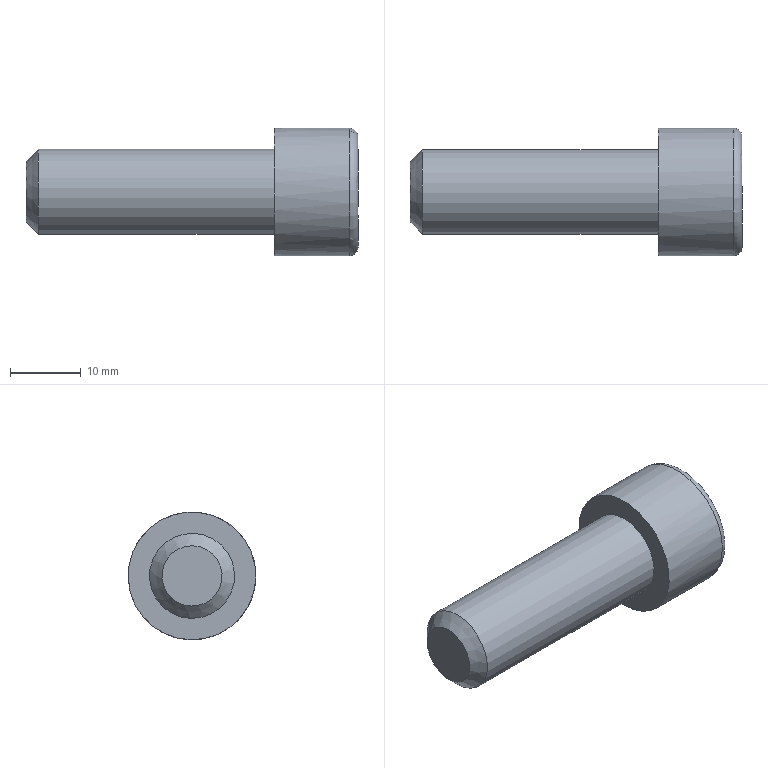Component | NX | 12_03_SCREW_M12X35_DIN912_2 | 1 solid | 14 faces | box 46.8 x 18 x 18 mm | volume 6372 mm3 | plane 10 | cylinder 2 | cone 1 | torus 1 | commonest cylinder face diameters 12 x1 18 x1
STEP:
#1=CARTESIAN_POINT('',(0.,0.,0.));
#2=DIRECTION('',(0.,0.,1.));
#3=DIRECTION('',(1.,0.,0.));
#4=AXIS2_PLACEMENT_3D('',#1,#2,#3);
#5=CARTESIAN_POINT('',(30.8,27.791,32.022));
#6=VERTEX_POINT('',#5);
#7=CARTESIAN_POINT('',(30.8,35.,35.));
#8=DIRECTION('',(1.,0.,0.));
#9=DIRECTION('',(0.,-0.9242,-0.3818));
#10=AXIS2_PLACEMENT_3D('',#7,#8,#9);
#11=CIRCLE('',#10,7.8);
#12=CARTESIAN_POINT('',(30.8,43.318,38.437));
#13=DIRECTION('',(-1.,-0.,-0.));
#14=DIRECTION('',(0.,-0.9242,-0.3818));
#15=AXIS2_PLACEMENT_3D('',#12,#13,#14);
#16=PLANE('',#15);
#17=CARTESIAN_POINT('',(16.8,0.));
#18=CARTESIAN_POINT('',(16.8,-13.51));
#19=CARTESIAN_POINT('',(5.1,-6.755));
#20=CARTESIAN_POINT('',(-6.6,0.));
#21=CARTESIAN_POINT('',(5.1,6.755));
#22=CARTESIAN_POINT('',(16.8,13.51));
#23=CARTESIAN_POINT('',(16.8,0.));
#24=(BOUNDED_CURVE()B_SPLINE_CURVE(2,(#17,#18,#19,#20,#21,#22,#23),.UNSPECIFIED.,.T.,.F.)B_SPLINE_CURVE_WITH_KNOTS((1,2,2,2,2,1),(-2.094,0.,2.094,4.189,6.283,8.378),.UNSPECIFIED.)CURVE()GEOMETRIC_REPRESENTATION_ITEM()RATIONAL_B_SPLINE_CURVE((1.,0.5,1.,0.5,1.,0.5,1.))REPRESENTATION_ITEM(''));
#25=(GEOMETRIC_REPRESENTATION_CONTEXT(2)PARAMETRIC_REPRESENTATION_CONTEXT()REPRESENTATION_CONTEXT('',''));
#26=DEFINITIONAL_REPRESENTATION('',(#24),#25);
#27=PCURVE('',#16,#26);
#28=CARTESIAN_POINT('',(29.6,35.,35.));
#29=DIRECTION('',(-1.,-0.,-0.));
#30=DIRECTION('',(0.,-0.9242,-0.3818));
#31=AXIS2_PLACEMENT_3D('',#28,#29,#30);
#32=TOROIDAL_SURFACE('',#31,7.8,1.2);
#33=CARTESIAN_POINT('',(6.283,4.712));
#34=DIRECTION('',(-1.,0.));
#35=VECTOR('',#34,1.);
#36=LINE('',#33,#35);
#37=(GEOMETRIC_REPRESENTATION_CONTEXT(2)PARAMETRIC_REPRESENTATION_CONTEXT()REPRESENTATION_CONTEXT('',''));
#38=DEFINITIONAL_REPRESENTATION('',(#36),#37);
#39=PCURVE('',#32,#38);
#40=SURFACE_CURVE('',#11,(#27,#39),.PCURVE_S1.);
#41=EDGE_CURVE('',#6,#6,#40,.T.);
#42=ORIENTED_EDGE('',*,*,#41,.T.);
#43=EDGE_LOOP('',(#42));
#44=FACE_BOUND('',#43,.T.);
#45=CARTESIAN_POINT('',(30.8,39.577,31.481));
#46=VERTEX_POINT('',#45);
#47=CARTESIAN_POINT('',(30.8,40.336,37.205));
#48=VERTEX_POINT('',#47);
#49=CARTESIAN_POINT('',(30.8,39.577,31.481));
#50=DIRECTION('',(0.,0.1314,0.9913));
#51=VECTOR('',#50,1.);
#52=LINE('',#49,#51);
#53=CARTESIAN_POINT('',(6.113,-5.));
#54=DIRECTION('',(-0.5,0.866));
#55=VECTOR('',#54,1.);
#56=LINE('',#53,#55);
#57=(GEOMETRIC_REPRESENTATION_CONTEXT(2)PARAMETRIC_REPRESENTATION_CONTEXT()REPRESENTATION_CONTEXT('',''));
#58=DEFINITIONAL_REPRESENTATION('',(#56),#57);
#59=PCURVE('',#16,#58);
#60=CARTESIAN_POINT('',(24.8,39.577,31.481));
#61=DIRECTION('',(0.,0.9913,-0.1314));
#62=DIRECTION('',(0.,-0.1314,-0.9913));
#63=AXIS2_PLACEMENT_3D('',#60,#61,#62);
#64=PLANE('',#63);
#65=CARTESIAN_POINT('',(0.,-6.));
#66=DIRECTION('',(-1.,0.));
#67=VECTOR('',#66,1.);
#68=LINE('',#65,#67);
#69=(GEOMETRIC_REPRESENTATION_CONTEXT(2)PARAMETRIC_REPRESENTATION_CONTEXT()REPRESENTATION_CONTEXT('',''));
#70=DEFINITIONAL_REPRESENTATION('',(#68),#69);
#71=PCURVE('',#64,#70);
#72=SURFACE_CURVE('',#52,(#59,#71),.PCURVE_S1.);
#73=EDGE_CURVE('',#46,#48,#72,.T.);
#74=ORIENTED_EDGE('',*,*,#73,.F.);
#75=CARTESIAN_POINT('',(30.8,34.241,29.277));
#76=VERTEX_POINT('',#75);
#77=CARTESIAN_POINT('',(30.8,34.241,29.277));
#78=DIRECTION('',(0.,0.9242,0.3818));
#79=VECTOR('',#78,1.);
#80=LINE('',#77,#79);
#81=CARTESIAN_POINT('',(11.887,-5.));
#82=DIRECTION('',(-1.,-0.));
#83=VECTOR('',#82,1.);
#84=LINE('',#81,#83);
#85=(GEOMETRIC_REPRESENTATION_CONTEXT(2)PARAMETRIC_REPRESENTATION_CONTEXT()REPRESENTATION_CONTEXT('',''));
#86=DEFINITIONAL_REPRESENTATION('',(#84),#85);
#87=PCURVE('',#16,#86);
#88=CARTESIAN_POINT('',(24.8,34.241,29.277));
#89=DIRECTION('',(0.,0.3818,-0.9242));
#90=DIRECTION('',(0.,-0.9242,-0.3818));
#91=AXIS2_PLACEMENT_3D('',#88,#89,#90);
#92=PLANE('',#91);
#93=CARTESIAN_POINT('',(0.,-6.));
#94=DIRECTION('',(-1.,0.));
#95=VECTOR('',#94,1.);
#96=LINE('',#93,#95);
#97=(GEOMETRIC_REPRESENTATION_CONTEXT(2)PARAMETRIC_REPRESENTATION_CONTEXT()REPRESENTATION_CONTEXT('',''));
#98=DEFINITIONAL_REPRESENTATION('',(#96),#97);
#99=PCURVE('',#92,#98);
#100=SURFACE_CURVE('',#80,(#87,#99),.PCURVE_S1.);
#101=EDGE_CURVE('',#76,#46,#100,.T.);
#102=ORIENTED_EDGE('',*,*,#101,.F.);
#103=CARTESIAN_POINT('',(30.8,29.664,32.795));
#104=VERTEX_POINT('',#103);
#105=CARTESIAN_POINT('',(30.8,29.664,32.795));
#106=DIRECTION('',(0.,0.7928,-0.6095));
#107=VECTOR('',#106,1.);
#108=LINE('',#105,#107);
#109=CARTESIAN_POINT('',(14.774,0.));
#110=DIRECTION('',(-0.5,-0.866));
#111=VECTOR('',#110,1.);
#112=LINE('',#109,#111);
#113=(GEOMETRIC_REPRESENTATION_CONTEXT(2)PARAMETRIC_REPRESENTATION_CONTEXT()REPRESENTATION_CONTEXT('',''));
#114=DEFINITIONAL_REPRESENTATION('',(#112),#113);
#115=PCURVE('',#16,#114);
#116=CARTESIAN_POINT('',(24.8,29.664,32.795));
#117=DIRECTION('',(0.,-0.6095,-0.7928));
#118=DIRECTION('',(0.,-0.7928,0.6095));
#119=AXIS2_PLACEMENT_3D('',#116,#117,#118);
#120=PLANE('',#119);
#121=CARTESIAN_POINT('',(0.,-6.));
#122=DIRECTION('',(-1.,0.));
#123=VECTOR('',#122,1.);
#124=LINE('',#121,#123);
#125=(GEOMETRIC_REPRESENTATION_CONTEXT(2)PARAMETRIC_REPRESENTATION_CONTEXT()REPRESENTATION_CONTEXT('',''));
#126=DEFINITIONAL_REPRESENTATION('',(#124),#125);
#127=PCURVE('',#120,#126);
#128=SURFACE_CURVE('',#108,(#115,#127),.PCURVE_S1.);
#129=EDGE_CURVE('',#104,#76,#128,.T.);
#130=ORIENTED_EDGE('',*,*,#129,.F.);
#131=CARTESIAN_POINT('',(30.8,30.423,38.519));
#132=VERTEX_POINT('',#131);
#133=CARTESIAN_POINT('',(30.8,30.423,38.519));
#134=DIRECTION('',(0.,-0.1314,-0.9913));
#135=VECTOR('',#134,1.);
#136=LINE('',#133,#135);
#137=CARTESIAN_POINT('',(11.887,5.));
#138=DIRECTION('',(0.5,-0.866));
#139=VECTOR('',#138,1.);
#140=LINE('',#137,#139);
#141=(GEOMETRIC_REPRESENTATION_CONTEXT(2)PARAMETRIC_REPRESENTATION_CONTEXT()REPRESENTATION_CONTEXT('',''));
#142=DEFINITIONAL_REPRESENTATION('',(#140),#141);
#143=PCURVE('',#16,#142);
#144=CARTESIAN_POINT('',(24.8,30.423,38.519));
#145=DIRECTION('',(0.,-0.9913,0.1314));
#146=DIRECTION('',(0.,0.1314,0.9913));
#147=AXIS2_PLACEMENT_3D('',#144,#145,#146);
#148=PLANE('',#147);
#149=CARTESIAN_POINT('',(0.,-6.));
#150=DIRECTION('',(-1.,0.));
#151=VECTOR('',#150,1.);
#152=LINE('',#149,#151);
#153=(GEOMETRIC_REPRESENTATION_CONTEXT(2)PARAMETRIC_REPRESENTATION_CONTEXT()REPRESENTATION_CONTEXT('',''));
#154=DEFINITIONAL_REPRESENTATION('',(#152),#153);
#155=PCURVE('',#148,#154);
#156=SURFACE_CURVE('',#136,(#143,#155),.PCURVE_S1.);
#157=EDGE_CURVE('',#132,#104,#156,.T.);
#158=ORIENTED_EDGE('',*,*,#157,.F.);
#159=CARTESIAN_POINT('',(30.8,35.759,40.723));
#160=VERTEX_POINT('',#159);
#161=CARTESIAN_POINT('',(30.8,35.759,40.723));
#162=DIRECTION('',(0.,-0.9242,-0.3818));
#163=VECTOR('',#162,1.);
#164=LINE('',#161,#163);
#165=CARTESIAN_POINT('',(6.113,5.));
#166=DIRECTION('',(1.,0.));
#167=VECTOR('',#166,1.);
#168=LINE('',#165,#167);
#169=(GEOMETRIC_REPRESENTATION_CONTEXT(2)PARAMETRIC_REPRESENTATION_CONTEXT()REPRESENTATION_CONTEXT('',''));
#170=DEFINITIONAL_REPRESENTATION('',(#168),#169);
#171=PCURVE('',#16,#170);
#172=CARTESIAN_POINT('',(24.8,35.759,40.723));
#173=DIRECTION('',(0.,-0.3818,0.9242));
#174=DIRECTION('',(0.,0.9242,0.3818));
#175=AXIS2_PLACEMENT_3D('',#172,#173,#174);
#176=PLANE('',#175);
#177=CARTESIAN_POINT('',(0.,-6.));
#178=DIRECTION('',(-1.,0.));
#179=VECTOR('',#178,1.);
#180=LINE('',#177,#179);
#181=(GEOMETRIC_REPRESENTATION_CONTEXT(2)PARAMETRIC_REPRESENTATION_CONTEXT()REPRESENTATION_CONTEXT('',''));
#182=DEFINITIONAL_REPRESENTATION('',(#180),#181);
#183=PCURVE('',#176,#182);
#184=SURFACE_CURVE('',#164,(#171,#183),.PCURVE_S1.);
#185=EDGE_CURVE('',#160,#132,#184,.T.);
#186=ORIENTED_EDGE('',*,*,#185,.F.);
#187=CARTESIAN_POINT('',(30.8,40.336,37.205));
#188=DIRECTION('',(0.,-0.7928,0.6095));
#189=VECTOR('',#188,1.);
#190=LINE('',#187,#189);
#191=CARTESIAN_POINT('',(3.226,0.));
#192=DIRECTION('',(0.5,0.866));
#193=VECTOR('',#192,1.);
#194=LINE('',#191,#193);
#195=(GEOMETRIC_REPRESENTATION_CONTEXT(2)PARAMETRIC_REPRESENTATION_CONTEXT()REPRESENTATION_CONTEXT('',''));
#196=DEFINITIONAL_REPRESENTATION('',(#194),#195);
#197=PCURVE('',#16,#196);
#198=CARTESIAN_POINT('',(24.8,40.336,37.205));
#199=DIRECTION('',(0.,0.6095,0.7928));
#200=DIRECTION('',(0.,0.7928,-0.6095));
#201=AXIS2_PLACEMENT_3D('',#198,#199,#200);
#202=PLANE('',#201);
#203=CARTESIAN_POINT('',(0.,-6.));
#204=DIRECTION('',(-1.,0.));
#205=VECTOR('',#204,1.);
#206=LINE('',#203,#205);
#207=(GEOMETRIC_REPRESENTATION_CONTEXT(2)PARAMETRIC_REPRESENTATION_CONTEXT()REPRESENTATION_CONTEXT('',''));
#208=DEFINITIONAL_REPRESENTATION('',(#206),#207);
#209=PCURVE('',#202,#208);
#210=SURFACE_CURVE('',#190,(#197,#209),.PCURVE_S1.);
#211=EDGE_CURVE('',#48,#160,#210,.T.);
#212=ORIENTED_EDGE('',*,*,#211,.F.);
#213=EDGE_LOOP('',(#74,#102,#130,#158,#186,#212));
#214=FACE_BOUND('',#213,.T.);
#215=ADVANCED_FACE('',(#44,#214),#16,.F.);
#216=CARTESIAN_POINT('',(-16.,38.928,36.623));
#217=VERTEX_POINT('',#216);
#218=CARTESIAN_POINT('',(-16.,35.,35.));
#219=DIRECTION('',(-1.,-0.,-0.));
#220=DIRECTION('',(-0.,0.9242,0.3818));
#221=AXIS2_PLACEMENT_3D('',#218,#219,#220);
#222=CIRCLE('',#221,4.25);
#223=CARTESIAN_POINT('',(-16.,35.,35.));
#224=DIRECTION('',(1.,0.,0.));
#225=DIRECTION('',(-0.,0.9242,0.3818));
#226=AXIS2_PLACEMENT_3D('',#223,#224,#225);
#227=PLANE('',#226);
#228=CARTESIAN_POINT('',(4.25,0.));
#229=CARTESIAN_POINT('',(4.25,-7.361));
#230=CARTESIAN_POINT('',(-2.125,-3.681));
#231=CARTESIAN_POINT('',(-8.5,-0.));
#232=CARTESIAN_POINT('',(-2.125,3.681));
#233=CARTESIAN_POINT('',(4.25,7.361));
#234=CARTESIAN_POINT('',(4.25,0.));
#235=(BOUNDED_CURVE()B_SPLINE_CURVE(2,(#228,#229,#230,#231,#232,#233,#234),.UNSPECIFIED.,.T.,.F.)B_SPLINE_CURVE_WITH_KNOTS((1,2,2,2,2,1),(-2.094,0.,2.094,4.189,6.283,8.378),.UNSPECIFIED.)CURVE()GEOMETRIC_REPRESENTATION_ITEM()RATIONAL_B_SPLINE_CURVE((1.,0.5,1.,0.5,1.,0.5,1.))REPRESENTATION_ITEM(''));
#236=(GEOMETRIC_REPRESENTATION_CONTEXT(2)PARAMETRIC_REPRESENTATION_CONTEXT()REPRESENTATION_CONTEXT('',''));
#237=DEFINITIONAL_REPRESENTATION('',(#235),#236);
#238=PCURVE('',#227,#237);
#239=CARTESIAN_POINT('',(-14.25,35.,35.));
#240=DIRECTION('',(1.,0.,0.));
#241=DIRECTION('',(-0.,0.9242,0.3818));
#242=AXIS2_PLACEMENT_3D('',#239,#240,#241);
#243=CONICAL_SURFACE('',#242,6.,0.7854);
#244=CARTESIAN_POINT('',(6.283,-1.75));
#245=DIRECTION('',(-1.,-0.));
#246=VECTOR('',#245,1.);
#247=LINE('',#244,#246);
#248=(GEOMETRIC_REPRESENTATION_CONTEXT(2)PARAMETRIC_REPRESENTATION_CONTEXT()REPRESENTATION_CONTEXT('',''));
#249=DEFINITIONAL_REPRESENTATION('',(#247),#248);
#250=PCURVE('',#243,#249);
#251=SURFACE_CURVE('',#222,(#238,#250),.PCURVE_S1.);
#252=EDGE_CURVE('',#217,#217,#251,.T.);
#253=ORIENTED_EDGE('',*,*,#252,.T.);
#254=EDGE_LOOP('',(#253));
#255=FACE_BOUND('',#254,.T.);
#256=ADVANCED_FACE('',(#255),#227,.F.);
#257=CARTESIAN_POINT('',(-14.25,40.545,37.291));
#258=VERTEX_POINT('',#257);
#259=CARTESIAN_POINT('',(-14.25,35.,35.));
#260=DIRECTION('',(1.,0.,0.));
#261=DIRECTION('',(-0.,0.9242,0.3818));
#262=AXIS2_PLACEMENT_3D('',#259,#260,#261);
#263=CIRCLE('',#262,6.);
#264=CARTESIAN_POINT('',(-16.,35.,35.));
#265=DIRECTION('',(1.,0.,0.));
#266=DIRECTION('',(-0.,0.9242,0.3818));
#267=AXIS2_PLACEMENT_3D('',#264,#265,#266);
#268=CYLINDRICAL_SURFACE('',#267,6.);
#269=CARTESIAN_POINT('',(0.,1.75));
#270=DIRECTION('',(1.,0.));
#271=VECTOR('',#270,1.);
#272=LINE('',#269,#271);
#273=(GEOMETRIC_REPRESENTATION_CONTEXT(2)PARAMETRIC_REPRESENTATION_CONTEXT()REPRESENTATION_CONTEXT('',''));
#274=DEFINITIONAL_REPRESENTATION('',(#272),#273);
#275=PCURVE('',#268,#274);
#276=CARTESIAN_POINT('',(0.,0.));
#277=DIRECTION('',(1.,-0.));
#278=VECTOR('',#277,1.);
#279=LINE('',#276,#278);
#280=(GEOMETRIC_REPRESENTATION_CONTEXT(2)PARAMETRIC_REPRESENTATION_CONTEXT()REPRESENTATION_CONTEXT('',''));
#281=DEFINITIONAL_REPRESENTATION('',(#279),#280);
#282=PCURVE('',#243,#281);
#283=SURFACE_CURVE('',#263,(#275,#282),.PCURVE_S1.);
#284=EDGE_CURVE('',#258,#258,#283,.T.);
#285=ORIENTED_EDGE('',*,*,#284,.T.);
#286=CARTESIAN_POINT('',(19.,40.545,37.291));
#287=VERTEX_POINT('',#286);
#288=CARTESIAN_POINT('',(-14.25,40.545,37.291));
#289=CARTESIAN_POINT('',(19.,40.545,37.291));
#290=B_SPLINE_CURVE_WITH_KNOTS('',1,(#288,#289),.UNSPECIFIED.,.F.,.F.,(2,2),(1.75,35.),.PIECEWISE_BEZIER_KNOTS.);
#291=CARTESIAN_POINT('',(6.283,0.));
#292=DIRECTION('',(0.,1.));
#293=VECTOR('',#292,1.);
#294=LINE('',#291,#293);
#295=(GEOMETRIC_REPRESENTATION_CONTEXT(2)PARAMETRIC_REPRESENTATION_CONTEXT()REPRESENTATION_CONTEXT('',''));
#296=DEFINITIONAL_REPRESENTATION('',(#294),#295);
#297=PCURVE('',#268,#296);
#298=CARTESIAN_POINT('',(0.,0.));
#299=DIRECTION('',(0.,1.));
#300=VECTOR('',#299,1.);
#301=LINE('',#298,#300);
#302=(GEOMETRIC_REPRESENTATION_CONTEXT(2)PARAMETRIC_REPRESENTATION_CONTEXT()REPRESENTATION_CONTEXT('',''));
#303=DEFINITIONAL_REPRESENTATION('',(#301),#302);
#304=PCURVE('',#268,#303);
#305=SEAM_CURVE('',#290,(#297,#304),.PCURVE_S1.);
#306=EDGE_CURVE('',#258,#287,#305,.T.);
#307=ORIENTED_EDGE('',*,*,#306,.T.);
#308=CARTESIAN_POINT('',(19.,35.,35.));
#309=DIRECTION('',(1.,0.,0.));
#310=DIRECTION('',(-0.,0.9242,0.3818));
#311=AXIS2_PLACEMENT_3D('',#308,#309,#310);
#312=CIRCLE('',#311,6.);
#313=CARTESIAN_POINT('',(0.,35.));
#314=DIRECTION('',(1.,0.));
#315=VECTOR('',#314,1.);
#316=LINE('',#313,#315);
#317=(GEOMETRIC_REPRESENTATION_CONTEXT(2)PARAMETRIC_REPRESENTATION_CONTEXT()REPRESENTATION_CONTEXT('',''));
#318=DEFINITIONAL_REPRESENTATION('',(#316),#317);
#319=PCURVE('',#268,#318);
#320=CARTESIAN_POINT('',(19.,40.545,37.291));
#321=DIRECTION('',(1.,0.,0.));
#322=DIRECTION('',(-0.,0.9242,0.3818));
#323=AXIS2_PLACEMENT_3D('',#320,#321,#322);
#324=PLANE('',#323);
#325=CARTESIAN_POINT('',(-6.,0.));
#326=DIRECTION('',(1.,0.));
#327=AXIS2_PLACEMENT_2D('',#325,#326);
#328=CIRCLE('',#327,6.);
#329=(GEOMETRIC_REPRESENTATION_CONTEXT(2)PARAMETRIC_REPRESENTATION_CONTEXT()REPRESENTATION_CONTEXT('',''));
#330=DEFINITIONAL_REPRESENTATION('',(#328),#329);
#331=PCURVE('',#324,#330);
#332=SURFACE_CURVE('',#312,(#319,#331),.PCURVE_S1.);
#333=EDGE_CURVE('',#287,#287,#332,.T.);
#334=ORIENTED_EDGE('',*,*,#333,.F.);
#335=ORIENTED_EDGE('',*,*,#306,.F.);
#336=EDGE_LOOP('',(#285,#307,#334,#335));
#337=FACE_BOUND('',#336,.T.);
#338=ADVANCED_FACE('',(#337),#268,.T.);
#339=CARTESIAN_POINT('',(19.,43.318,38.437));
#340=VERTEX_POINT('',#339);
#341=CARTESIAN_POINT('',(19.,35.,35.));
#342=DIRECTION('',(1.,0.,0.));
#343=DIRECTION('',(-0.,0.9242,0.3818));
#344=AXIS2_PLACEMENT_3D('',#341,#342,#343);
#345=CIRCLE('',#344,9.);
#346=CARTESIAN_POINT('',(-6.,0.));
#347=DIRECTION('',(1.,0.));
#348=AXIS2_PLACEMENT_2D('',#346,#347);
#349=CIRCLE('',#348,9.);
#350=(GEOMETRIC_REPRESENTATION_CONTEXT(2)PARAMETRIC_REPRESENTATION_CONTEXT()REPRESENTATION_CONTEXT('',''));
#351=DEFINITIONAL_REPRESENTATION('',(#349),#350);
#352=PCURVE('',#324,#351);
#353=CARTESIAN_POINT('',(-16.,35.,35.));
#354=DIRECTION('',(1.,0.,0.));
#355=DIRECTION('',(-0.,0.9242,0.3818));
#356=AXIS2_PLACEMENT_3D('',#353,#354,#355);
#357=CYLINDRICAL_SURFACE('',#356,9.);
#358=CARTESIAN_POINT('',(0.,35.));
#359=DIRECTION('',(1.,0.));
#360=VECTOR('',#359,1.);
#361=LINE('',#358,#360);
#362=(GEOMETRIC_REPRESENTATION_CONTEXT(2)PARAMETRIC_REPRESENTATION_CONTEXT()REPRESENTATION_CONTEXT('',''));
#363=DEFINITIONAL_REPRESENTATION('',(#361),#362);
#364=PCURVE('',#357,#363);
#365=SURFACE_CURVE('',#345,(#352,#364),.PCURVE_S1.);
#366=EDGE_CURVE('',#340,#340,#365,.T.);
#367=ORIENTED_EDGE('',*,*,#366,.F.);
#368=EDGE_LOOP('',(#367));
#369=FACE_BOUND('',#368,.T.);
#370=ORIENTED_EDGE('',*,*,#333,.T.);
#371=EDGE_LOOP('',(#370));
#372=FACE_BOUND('',#371,.T.);
#373=ADVANCED_FACE('',(#369,#372),#324,.F.);
#374=CARTESIAN_POINT('',(29.6,26.682,31.563));
#375=VERTEX_POINT('',#374);
#376=CARTESIAN_POINT('',(29.6,43.318,38.437));
#377=VERTEX_POINT('',#376);
#378=CARTESIAN_POINT('',(29.6,35.,35.));
#379=DIRECTION('',(-1.,-0.,-0.));
#380=DIRECTION('',(0.,-0.9242,-0.3818));
#381=AXIS2_PLACEMENT_3D('',#378,#379,#380);
#382=CIRCLE('',#381,9.);
#383=CARTESIAN_POINT('',(3.142,45.6));
#384=DIRECTION('',(-1.,0.));
#385=VECTOR('',#384,1.);
#386=LINE('',#383,#385);
#387=(GEOMETRIC_REPRESENTATION_CONTEXT(2)PARAMETRIC_REPRESENTATION_CONTEXT()REPRESENTATION_CONTEXT('',''));
#388=DEFINITIONAL_REPRESENTATION('',(#386),#387);
#389=PCURVE('',#357,#388);
#390=CARTESIAN_POINT('',(0.,6.283));
#391=CARTESIAN_POINT('',(0.0476,6.283));
#392=CARTESIAN_POINT('',(0.1428,6.283));
#393=CARTESIAN_POINT('',(0.2856,6.283));
#394=CARTESIAN_POINT('',(0.4284,6.283));
#395=CARTESIAN_POINT('',(0.5712,6.283));
#396=CARTESIAN_POINT('',(0.714,6.283));
#397=CARTESIAN_POINT('',(0.8568,6.283));
#398=CARTESIAN_POINT('',(0.9996,6.283));
#399=CARTESIAN_POINT('',(1.142,6.283));
#400=CARTESIAN_POINT('',(1.285,6.283));
#401=CARTESIAN_POINT('',(1.428,6.283));
#402=CARTESIAN_POINT('',(1.571,6.283));
#403=CARTESIAN_POINT('',(1.714,6.283));
#404=CARTESIAN_POINT('',(1.856,6.283));
#405=CARTESIAN_POINT('',(1.999,6.283));
#406=CARTESIAN_POINT('',(2.142,6.283));
#407=CARTESIAN_POINT('',(2.285,6.283));
#408=CARTESIAN_POINT('',(2.428,6.283));
#409=CARTESIAN_POINT('',(2.57,6.283));
#410=CARTESIAN_POINT('',(2.713,6.283));
#411=CARTESIAN_POINT('',(2.856,6.283));
#412=CARTESIAN_POINT('',(2.999,6.283));
#413=CARTESIAN_POINT('',(3.094,6.283));
#414=CARTESIAN_POINT('',(3.142,6.283));
#415=B_SPLINE_CURVE_WITH_KNOTS('',3,(#390,#391,#392,#393,#394,#395,#396,#397,#398,#399,#400,#401,#402,#403,#404,#405,#406,#407,#408,#409,#410,#411,#412,#413,#414),.UNSPECIFIED.,.F.,.F.,(4,1,1,1,1,1,1,1,1,1,1,1,1,1,1,1,1,1,1,1,1,1,4),(0.,0.1428,0.2856,0.4284,0.5712,0.714,0.8568,0.9996,1.142,1.285,1.428,1.571,1.714,1.856,1.999,2.142,2.285,2.428,2.57,2.713,2.856,2.999,3.142),.QUASI_UNIFORM_KNOTS.);
#416=(GEOMETRIC_REPRESENTATION_CONTEXT(2)PARAMETRIC_REPRESENTATION_CONTEXT()REPRESENTATION_CONTEXT('',''));
#417=DEFINITIONAL_REPRESENTATION('',(#415),#416);
#418=PCURVE('',#32,#417);
#419=SURFACE_CURVE('',#382,(#389,#418),.PCURVE_S1.);
#420=EDGE_CURVE('',#375,#377,#419,.T.);
#421=ORIENTED_EDGE('',*,*,#420,.T.);
#422=CARTESIAN_POINT('',(19.,43.318,38.437));
#423=CARTESIAN_POINT('',(29.6,43.318,38.437));
#424=B_SPLINE_CURVE_WITH_KNOTS('',1,(#422,#423),.UNSPECIFIED.,.F.,.F.,(2,2),(35.,45.6),.PIECEWISE_BEZIER_KNOTS.);
#425=CARTESIAN_POINT('',(0.,0.));
#426=DIRECTION('',(0.,1.));
#427=VECTOR('',#426,1.);
#428=LINE('',#425,#427);
#429=(GEOMETRIC_REPRESENTATION_CONTEXT(2)PARAMETRIC_REPRESENTATION_CONTEXT()REPRESENTATION_CONTEXT('',''));
#430=DEFINITIONAL_REPRESENTATION('',(#428),#429);
#431=PCURVE('',#357,#430);
#432=CARTESIAN_POINT('',(6.283,0.));
#433=DIRECTION('',(0.,1.));
#434=VECTOR('',#433,1.);
#435=LINE('',#432,#434);
#436=(GEOMETRIC_REPRESENTATION_CONTEXT(2)PARAMETRIC_REPRESENTATION_CONTEXT()REPRESENTATION_CONTEXT('',''));
#437=DEFINITIONAL_REPRESENTATION('',(#435),#436);
#438=PCURVE('',#357,#437);
#439=SEAM_CURVE('',#424,(#431,#438),.PCURVE_S1.);
#440=EDGE_CURVE('',#340,#377,#439,.T.);
#441=ORIENTED_EDGE('',*,*,#440,.F.);
#442=ORIENTED_EDGE('',*,*,#366,.T.);
#443=ORIENTED_EDGE('',*,*,#440,.T.);
#444=CARTESIAN_POINT('',(29.6,35.,35.));
#445=DIRECTION('',(-1.,-0.,-0.));
#446=DIRECTION('',(0.,-0.9242,-0.3818));
#447=AXIS2_PLACEMENT_3D('',#444,#445,#446);
#448=CIRCLE('',#447,9.);
#449=CARTESIAN_POINT('',(9.425,45.6));
#450=DIRECTION('',(-1.,0.));
#451=VECTOR('',#450,1.);
#452=LINE('',#449,#451);
#453=(GEOMETRIC_REPRESENTATION_CONTEXT(2)PARAMETRIC_REPRESENTATION_CONTEXT()REPRESENTATION_CONTEXT('',''));
#454=DEFINITIONAL_REPRESENTATION('',(#452),#453);
#455=PCURVE('',#357,#454);
#456=CARTESIAN_POINT('',(0.,6.283));
#457=DIRECTION('',(1.,0.));
#458=VECTOR('',#457,1.);
#459=LINE('',#456,#458);
#460=(GEOMETRIC_REPRESENTATION_CONTEXT(2)PARAMETRIC_REPRESENTATION_CONTEXT()REPRESENTATION_CONTEXT('',''));
#461=DEFINITIONAL_REPRESENTATION('',(#459),#460);
#462=PCURVE('',#32,#461);
#463=SURFACE_CURVE('',#448,(#455,#462),.PCURVE_S1.);
#464=EDGE_CURVE('',#377,#375,#463,.T.);
#465=ORIENTED_EDGE('',*,*,#464,.T.);
#466=EDGE_LOOP('',(#421,#441,#442,#443,#465));
#467=FACE_BOUND('',#466,.T.);
#468=ADVANCED_FACE('',(#467),#357,.T.);
#469=ORIENTED_EDGE('',*,*,#101,.T.);
#470=CARTESIAN_POINT('',(24.8,39.577,31.481));
#471=VERTEX_POINT('',#470);
#472=CARTESIAN_POINT('',(24.8,39.577,31.481));
#473=DIRECTION('',(-1.,0.,0.));
#474=VECTOR('',#473,1.);
#475=LINE('',#472,#474);
#476=CARTESIAN_POINT('',(-5.774,0.));
#477=DIRECTION('',(0.,1.));
#478=VECTOR('',#477,1.);
#479=LINE('',#476,#478);
#480=(GEOMETRIC_REPRESENTATION_CONTEXT(2)PARAMETRIC_REPRESENTATION_CONTEXT()REPRESENTATION_CONTEXT('',''));
#481=DEFINITIONAL_REPRESENTATION('',(#479),#480);
#482=PCURVE('',#92,#481);
#483=CARTESIAN_POINT('',(-0.,0.));
#484=DIRECTION('',(0.,1.));
#485=VECTOR('',#484,1.);
#486=LINE('',#483,#485);
#487=(GEOMETRIC_REPRESENTATION_CONTEXT(2)PARAMETRIC_REPRESENTATION_CONTEXT()REPRESENTATION_CONTEXT('',''));
#488=DEFINITIONAL_REPRESENTATION('',(#486),#487);
#489=PCURVE('',#64,#488);
#490=SURFACE_CURVE('',#475,(#482,#489),.PCURVE_S1.);
#491=EDGE_CURVE('',#46,#471,#490,.T.);
#492=ORIENTED_EDGE('',*,*,#491,.T.);
#493=CARTESIAN_POINT('',(24.8,34.241,29.277));
#494=VERTEX_POINT('',#493);
#495=CARTESIAN_POINT('',(24.8,34.241,29.277));
#496=DIRECTION('',(0.,-0.9242,-0.3818));
#497=VECTOR('',#496,1.);
#498=LINE('',#495,#497);
#499=CARTESIAN_POINT('',(0.,0.));
#500=DIRECTION('',(1.,0.));
#501=VECTOR('',#500,1.);
#502=LINE('',#499,#501);
#503=(GEOMETRIC_REPRESENTATION_CONTEXT(2)PARAMETRIC_REPRESENTATION_CONTEXT()REPRESENTATION_CONTEXT('',''));
#504=DEFINITIONAL_REPRESENTATION('',(#502),#503);
#505=PCURVE('',#92,#504);
#506=CARTESIAN_POINT('',(24.8,35.,35.));
#507=DIRECTION('',(1.,0.,0.));
#508=DIRECTION('',(0.,0.9242,0.3818));
#509=AXIS2_PLACEMENT_3D('',#506,#507,#508);
#510=PLANE('',#509);
#511=CARTESIAN_POINT('',(-2.887,-5.));
#512=DIRECTION('',(-1.,0.));
#513=VECTOR('',#512,1.);
#514=LINE('',#511,#513);
#515=(GEOMETRIC_REPRESENTATION_CONTEXT(2)PARAMETRIC_REPRESENTATION_CONTEXT()REPRESENTATION_CONTEXT('',''));
#516=DEFINITIONAL_REPRESENTATION('',(#514),#515);
#517=PCURVE('',#510,#516);
#518=SURFACE_CURVE('',#498,(#505,#517),.PCURVE_S1.);
#519=EDGE_CURVE('',#471,#494,#518,.T.);
#520=ORIENTED_EDGE('',*,*,#519,.T.);
#521=CARTESIAN_POINT('',(24.8,34.241,29.277));
#522=DIRECTION('',(-1.,0.,0.));
#523=VECTOR('',#522,1.);
#524=LINE('',#521,#523);
#525=CARTESIAN_POINT('',(0.,0.));
#526=DIRECTION('',(0.,1.));
#527=VECTOR('',#526,1.);
#528=LINE('',#525,#527);
#529=(GEOMETRIC_REPRESENTATION_CONTEXT(2)PARAMETRIC_REPRESENTATION_CONTEXT()REPRESENTATION_CONTEXT('',''));
#530=DEFINITIONAL_REPRESENTATION('',(#528),#529);
#531=PCURVE('',#92,#530);
#532=CARTESIAN_POINT('',(-5.774,0.));
#533=DIRECTION('',(0.,1.));
#534=VECTOR('',#533,1.);
#535=LINE('',#532,#534);
#536=(GEOMETRIC_REPRESENTATION_CONTEXT(2)PARAMETRIC_REPRESENTATION_CONTEXT()REPRESENTATION_CONTEXT('',''));
#537=DEFINITIONAL_REPRESENTATION('',(#535),#536);
#538=PCURVE('',#120,#537);
#539=SURFACE_CURVE('',#524,(#531,#538),.PCURVE_S1.);
#540=EDGE_CURVE('',#76,#494,#539,.T.);
#541=ORIENTED_EDGE('',*,*,#540,.F.);
#542=EDGE_LOOP('',(#469,#492,#520,#541));
#543=FACE_BOUND('',#542,.T.);
#544=ADVANCED_FACE('',(#543),#92,.F.);
#545=ORIENTED_EDGE('',*,*,#73,.T.);
#546=CARTESIAN_POINT('',(24.8,40.336,37.205));
#547=VERTEX_POINT('',#546);
#548=CARTESIAN_POINT('',(24.8,40.336,37.205));
#549=DIRECTION('',(-1.,0.,0.));
#550=VECTOR('',#549,1.);
#551=LINE('',#548,#550);
#552=CARTESIAN_POINT('',(-5.774,0.));
#553=DIRECTION('',(0.,1.));
#554=VECTOR('',#553,1.);
#555=LINE('',#552,#554);
#556=(GEOMETRIC_REPRESENTATION_CONTEXT(2)PARAMETRIC_REPRESENTATION_CONTEXT()REPRESENTATION_CONTEXT('',''));
#557=DEFINITIONAL_REPRESENTATION('',(#555),#556);
#558=PCURVE('',#64,#557);
#559=CARTESIAN_POINT('',(0.,0.));
#560=DIRECTION('',(0.,1.));
#561=VECTOR('',#560,1.);
#562=LINE('',#559,#561);
#563=(GEOMETRIC_REPRESENTATION_CONTEXT(2)PARAMETRIC_REPRESENTATION_CONTEXT()REPRESENTATION_CONTEXT('',''));
#564=DEFINITIONAL_REPRESENTATION('',(#562),#563);
#565=PCURVE('',#202,#564);
#566=SURFACE_CURVE('',#551,(#558,#565),.PCURVE_S1.);
#567=EDGE_CURVE('',#48,#547,#566,.T.);
#568=ORIENTED_EDGE('',*,*,#567,.T.);
#569=CARTESIAN_POINT('',(24.8,39.577,31.481));
#570=DIRECTION('',(0.,-0.1314,-0.9913));
#571=VECTOR('',#570,1.);
#572=LINE('',#569,#571);
#573=CARTESIAN_POINT('',(0.,0.));
#574=DIRECTION('',(1.,0.));
#575=VECTOR('',#574,1.);
#576=LINE('',#573,#575);
#577=(GEOMETRIC_REPRESENTATION_CONTEXT(2)PARAMETRIC_REPRESENTATION_CONTEXT()REPRESENTATION_CONTEXT('',''));
#578=DEFINITIONAL_REPRESENTATION('',(#576),#577);
#579=PCURVE('',#64,#578);
#580=CARTESIAN_POINT('',(2.887,-5.));
#581=DIRECTION('',(-0.5,-0.866));
#582=VECTOR('',#581,1.);
#583=LINE('',#580,#582);
#584=(GEOMETRIC_REPRESENTATION_CONTEXT(2)PARAMETRIC_REPRESENTATION_CONTEXT()REPRESENTATION_CONTEXT('',''));
#585=DEFINITIONAL_REPRESENTATION('',(#583),#584);
#586=PCURVE('',#510,#585);
#587=SURFACE_CURVE('',#572,(#579,#586),.PCURVE_S1.);
#588=EDGE_CURVE('',#547,#471,#587,.T.);
#589=ORIENTED_EDGE('',*,*,#588,.T.);
#590=ORIENTED_EDGE('',*,*,#491,.F.);
#591=EDGE_LOOP('',(#545,#568,#589,#590));
#592=FACE_BOUND('',#591,.T.);
#593=ADVANCED_FACE('',(#592),#64,.F.);
#594=ORIENTED_EDGE('',*,*,#211,.T.);
#595=CARTESIAN_POINT('',(24.8,35.759,40.723));
#596=VERTEX_POINT('',#595);
#597=CARTESIAN_POINT('',(24.8,35.759,40.723));
#598=DIRECTION('',(-1.,0.,0.));
#599=VECTOR('',#598,1.);
#600=LINE('',#597,#599);
#601=CARTESIAN_POINT('',(-5.774,0.));
#602=DIRECTION('',(0.,1.));
#603=VECTOR('',#602,1.);
#604=LINE('',#601,#603);
#605=(GEOMETRIC_REPRESENTATION_CONTEXT(2)PARAMETRIC_REPRESENTATION_CONTEXT()REPRESENTATION_CONTEXT('',''));
#606=DEFINITIONAL_REPRESENTATION('',(#604),#605);
#607=PCURVE('',#202,#606);
#608=CARTESIAN_POINT('',(0.,0.));
#609=DIRECTION('',(0.,1.));
#610=VECTOR('',#609,1.);
#611=LINE('',#608,#610);
#612=(GEOMETRIC_REPRESENTATION_CONTEXT(2)PARAMETRIC_REPRESENTATION_CONTEXT()REPRESENTATION_CONTEXT('',''));
#613=DEFINITIONAL_REPRESENTATION('',(#611),#612);
#614=PCURVE('',#176,#613);
#615=SURFACE_CURVE('',#600,(#607,#614),.PCURVE_S1.);
#616=EDGE_CURVE('',#160,#596,#615,.T.);
#617=ORIENTED_EDGE('',*,*,#616,.T.);
#618=CARTESIAN_POINT('',(24.8,40.336,37.205));
#619=DIRECTION('',(0.,0.7928,-0.6095));
#620=VECTOR('',#619,1.);
#621=LINE('',#618,#620);
#622=CARTESIAN_POINT('',(0.,0.));
#623=DIRECTION('',(1.,0.));
#624=VECTOR('',#623,1.);
#625=LINE('',#622,#624);
#626=(GEOMETRIC_REPRESENTATION_CONTEXT(2)PARAMETRIC_REPRESENTATION_CONTEXT()REPRESENTATION_CONTEXT('',''));
#627=DEFINITIONAL_REPRESENTATION('',(#625),#626);
#628=PCURVE('',#202,#627);
#629=CARTESIAN_POINT('',(5.774,0.));
#630=DIRECTION('',(0.5,-0.866));
#631=VECTOR('',#630,1.);
#632=LINE('',#629,#631);
#633=(GEOMETRIC_REPRESENTATION_CONTEXT(2)PARAMETRIC_REPRESENTATION_CONTEXT()REPRESENTATION_CONTEXT('',''));
#634=DEFINITIONAL_REPRESENTATION('',(#632),#633);
#635=PCURVE('',#510,#634);
#636=SURFACE_CURVE('',#621,(#628,#635),.PCURVE_S1.);
#637=EDGE_CURVE('',#596,#547,#636,.T.);
#638=ORIENTED_EDGE('',*,*,#637,.T.);
#639=ORIENTED_EDGE('',*,*,#567,.F.);
#640=EDGE_LOOP('',(#594,#617,#638,#639));
#641=FACE_BOUND('',#640,.T.);
#642=ADVANCED_FACE('',(#641),#202,.F.);
#643=ORIENTED_EDGE('',*,*,#185,.T.);
#644=CARTESIAN_POINT('',(24.8,30.423,38.519));
#645=VERTEX_POINT('',#644);
#646=CARTESIAN_POINT('',(24.8,30.423,38.519));
#647=DIRECTION('',(-1.,0.,0.));
#648=VECTOR('',#647,1.);
#649=LINE('',#646,#648);
#650=CARTESIAN_POINT('',(-5.774,0.));
#651=DIRECTION('',(0.,1.));
#652=VECTOR('',#651,1.);
#653=LINE('',#650,#652);
#654=(GEOMETRIC_REPRESENTATION_CONTEXT(2)PARAMETRIC_REPRESENTATION_CONTEXT()REPRESENTATION_CONTEXT('',''));
#655=DEFINITIONAL_REPRESENTATION('',(#653),#654);
#656=PCURVE('',#176,#655);
#657=CARTESIAN_POINT('',(0.,0.));
#658=DIRECTION('',(0.,1.));
#659=VECTOR('',#658,1.);
#660=LINE('',#657,#659);
#661=(GEOMETRIC_REPRESENTATION_CONTEXT(2)PARAMETRIC_REPRESENTATION_CONTEXT()REPRESENTATION_CONTEXT('',''));
#662=DEFINITIONAL_REPRESENTATION('',(#660),#661);
#663=PCURVE('',#148,#662);
#664=SURFACE_CURVE('',#649,(#656,#663),.PCURVE_S1.);
#665=EDGE_CURVE('',#132,#645,#664,.T.);
#666=ORIENTED_EDGE('',*,*,#665,.T.);
#667=CARTESIAN_POINT('',(24.8,35.759,40.723));
#668=DIRECTION('',(0.,0.9242,0.3818));
#669=VECTOR('',#668,1.);
#670=LINE('',#667,#669);
#671=CARTESIAN_POINT('',(0.,0.));
#672=DIRECTION('',(1.,0.));
#673=VECTOR('',#672,1.);
#674=LINE('',#671,#673);
#675=(GEOMETRIC_REPRESENTATION_CONTEXT(2)PARAMETRIC_REPRESENTATION_CONTEXT()REPRESENTATION_CONTEXT('',''));
#676=DEFINITIONAL_REPRESENTATION('',(#674),#675);
#677=PCURVE('',#176,#676);
#678=CARTESIAN_POINT('',(2.887,5.));
#679=DIRECTION('',(1.,-0.));
#680=VECTOR('',#679,1.);
#681=LINE('',#678,#680);
#682=(GEOMETRIC_REPRESENTATION_CONTEXT(2)PARAMETRIC_REPRESENTATION_CONTEXT()REPRESENTATION_CONTEXT('',''));
#683=DEFINITIONAL_REPRESENTATION('',(#681),#682);
#684=PCURVE('',#510,#683);
#685=SURFACE_CURVE('',#670,(#677,#684),.PCURVE_S1.);
#686=EDGE_CURVE('',#645,#596,#685,.T.);
#687=ORIENTED_EDGE('',*,*,#686,.T.);
#688=ORIENTED_EDGE('',*,*,#616,.F.);
#689=EDGE_LOOP('',(#643,#666,#687,#688));
#690=FACE_BOUND('',#689,.T.);
#691=ADVANCED_FACE('',(#690),#176,.F.);
#692=ORIENTED_EDGE('',*,*,#157,.T.);
#693=CARTESIAN_POINT('',(24.8,29.664,32.795));
#694=VERTEX_POINT('',#693);
#695=CARTESIAN_POINT('',(24.8,29.664,32.795));
#696=DIRECTION('',(-1.,0.,0.));
#697=VECTOR('',#696,1.);
#698=LINE('',#695,#697);
#699=CARTESIAN_POINT('',(-5.774,0.));
#700=DIRECTION('',(0.,1.));
#701=VECTOR('',#700,1.);
#702=LINE('',#699,#701);
#703=(GEOMETRIC_REPRESENTATION_CONTEXT(2)PARAMETRIC_REPRESENTATION_CONTEXT()REPRESENTATION_CONTEXT('',''));
#704=DEFINITIONAL_REPRESENTATION('',(#702),#703);
#705=PCURVE('',#148,#704);
#706=CARTESIAN_POINT('',(0.,0.));
#707=DIRECTION('',(0.,1.));
#708=VECTOR('',#707,1.);
#709=LINE('',#706,#708);
#710=(GEOMETRIC_REPRESENTATION_CONTEXT(2)PARAMETRIC_REPRESENTATION_CONTEXT()REPRESENTATION_CONTEXT('',''));
#711=DEFINITIONAL_REPRESENTATION('',(#709),#710);
#712=PCURVE('',#120,#711);
#713=SURFACE_CURVE('',#698,(#705,#712),.PCURVE_S1.);
#714=EDGE_CURVE('',#104,#694,#713,.T.);
#715=ORIENTED_EDGE('',*,*,#714,.T.);
#716=CARTESIAN_POINT('',(24.8,30.423,38.519));
#717=DIRECTION('',(0.,0.1314,0.9913));
#718=VECTOR('',#717,1.);
#719=LINE('',#716,#718);
#720=CARTESIAN_POINT('',(0.,0.));
#721=DIRECTION('',(1.,0.));
#722=VECTOR('',#721,1.);
#723=LINE('',#720,#722);
#724=(GEOMETRIC_REPRESENTATION_CONTEXT(2)PARAMETRIC_REPRESENTATION_CONTEXT()REPRESENTATION_CONTEXT('',''));
#725=DEFINITIONAL_REPRESENTATION('',(#723),#724);
#726=PCURVE('',#148,#725);
#727=CARTESIAN_POINT('',(-2.887,5.));
#728=DIRECTION('',(0.5,0.866));
#729=VECTOR('',#728,1.);
#730=LINE('',#727,#729);
#731=(GEOMETRIC_REPRESENTATION_CONTEXT(2)PARAMETRIC_REPRESENTATION_CONTEXT()REPRESENTATION_CONTEXT('',''));
#732=DEFINITIONAL_REPRESENTATION('',(#730),#731);
#733=PCURVE('',#510,#732);
#734=SURFACE_CURVE('',#719,(#726,#733),.PCURVE_S1.);
#735=EDGE_CURVE('',#694,#645,#734,.T.);
#736=ORIENTED_EDGE('',*,*,#735,.T.);
#737=ORIENTED_EDGE('',*,*,#665,.F.);
#738=EDGE_LOOP('',(#692,#715,#736,#737));
#739=FACE_BOUND('',#738,.T.);
#740=ADVANCED_FACE('',(#739),#148,.F.);
#741=ORIENTED_EDGE('',*,*,#129,.T.);
#742=ORIENTED_EDGE('',*,*,#540,.T.);
#743=CARTESIAN_POINT('',(24.8,29.664,32.795));
#744=DIRECTION('',(0.,-0.7928,0.6095));
#745=VECTOR('',#744,1.);
#746=LINE('',#743,#745);
#747=CARTESIAN_POINT('',(0.,0.));
#748=DIRECTION('',(1.,0.));
#749=VECTOR('',#748,1.);
#750=LINE('',#747,#749);
#751=(GEOMETRIC_REPRESENTATION_CONTEXT(2)PARAMETRIC_REPRESENTATION_CONTEXT()REPRESENTATION_CONTEXT('',''));
#752=DEFINITIONAL_REPRESENTATION('',(#750),#751);
#753=PCURVE('',#120,#752);
#754=CARTESIAN_POINT('',(-5.774,0.));
#755=DIRECTION('',(-0.5,0.866));
#756=VECTOR('',#755,1.);
#757=LINE('',#754,#756);
#758=(GEOMETRIC_REPRESENTATION_CONTEXT(2)PARAMETRIC_REPRESENTATION_CONTEXT()REPRESENTATION_CONTEXT('',''));
#759=DEFINITIONAL_REPRESENTATION('',(#757),#758);
#760=PCURVE('',#510,#759);
#761=SURFACE_CURVE('',#746,(#753,#760),.PCURVE_S1.);
#762=EDGE_CURVE('',#494,#694,#761,.T.);
#763=ORIENTED_EDGE('',*,*,#762,.T.);
#764=ORIENTED_EDGE('',*,*,#714,.F.);
#765=EDGE_LOOP('',(#741,#742,#763,#764));
#766=FACE_BOUND('',#765,.T.);
#767=ADVANCED_FACE('',(#766),#120,.F.);
#768=ORIENTED_EDGE('',*,*,#519,.F.);
#769=ORIENTED_EDGE('',*,*,#588,.F.);
#770=ORIENTED_EDGE('',*,*,#637,.F.);
#771=ORIENTED_EDGE('',*,*,#686,.F.);
#772=ORIENTED_EDGE('',*,*,#735,.F.);
#773=ORIENTED_EDGE('',*,*,#762,.F.);
#774=EDGE_LOOP('',(#768,#769,#770,#771,#772,#773));
#775=FACE_BOUND('',#774,.T.);
#776=ADVANCED_FACE('',(#775),#510,.T.);
#777=ORIENTED_EDGE('',*,*,#252,.F.);
#778=CARTESIAN_POINT('',(-16.,38.928,36.623));
#779=CARTESIAN_POINT('',(-14.25,40.545,37.291));
#780=B_SPLINE_CURVE_WITH_KNOTS('',1,(#778,#779),.UNSPECIFIED.,.F.,.F.,(2,2),(-2.475,-0.),.PIECEWISE_BEZIER_KNOTS.);
#781=CARTESIAN_POINT('',(6.283,0.));
#782=DIRECTION('',(0.,1.));
#783=VECTOR('',#782,1.);
#784=LINE('',#781,#783);
#785=(GEOMETRIC_REPRESENTATION_CONTEXT(2)PARAMETRIC_REPRESENTATION_CONTEXT()REPRESENTATION_CONTEXT('',''));
#786=DEFINITIONAL_REPRESENTATION('',(#784),#785);
#787=PCURVE('',#243,#786);
#788=CARTESIAN_POINT('',(0.,0.));
#789=DIRECTION('',(0.,1.));
#790=VECTOR('',#789,1.);
#791=LINE('',#788,#790);
#792=(GEOMETRIC_REPRESENTATION_CONTEXT(2)PARAMETRIC_REPRESENTATION_CONTEXT()REPRESENTATION_CONTEXT('',''));
#793=DEFINITIONAL_REPRESENTATION('',(#791),#792);
#794=PCURVE('',#243,#793);
#795=SEAM_CURVE('',#780,(#787,#794),.PCURVE_S1.);
#796=EDGE_CURVE('',#217,#258,#795,.T.);
#797=ORIENTED_EDGE('',*,*,#796,.T.);
#798=ORIENTED_EDGE('',*,*,#284,.F.);
#799=ORIENTED_EDGE('',*,*,#796,.F.);
#800=EDGE_LOOP('',(#777,#797,#798,#799));
#801=FACE_BOUND('',#800,.T.);
#802=ADVANCED_FACE('',(#801),#243,.T.);
#803=ORIENTED_EDGE('',*,*,#420,.F.);
#804=CARTESIAN_POINT('',(30.8,27.791,32.022));
#805=CARTESIAN_POINT('',(30.8,27.495,31.899));
#806=CARTESIAN_POINT('',(30.698,27.206,31.78));
#807=CARTESIAN_POINT('',(30.502,26.957,31.677));
#808=CARTESIAN_POINT('',(30.233,26.776,31.602));
#809=CARTESIAN_POINT('',(29.921,26.682,31.563));
#810=CARTESIAN_POINT('',(29.6,26.682,31.563));
#811=(BOUNDED_CURVE()B_SPLINE_CURVE(6,(#804,#805,#806,#807,#808,#809,#810),.UNSPECIFIED.,.F.,.F.)B_SPLINE_CURVE_WITH_KNOTS((7,7),(4.712,6.283),.PIECEWISE_BEZIER_KNOTS.)CURVE()GEOMETRIC_REPRESENTATION_ITEM()RATIONAL_B_SPLINE_CURVE((1.031,1.01,0.9979,0.994,0.9979,1.01,1.031))REPRESENTATION_ITEM(''));
#812=CARTESIAN_POINT('',(0.,0.));
#813=DIRECTION('',(0.,1.));
#814=VECTOR('',#813,1.);
#815=LINE('',#812,#814);
#816=(GEOMETRIC_REPRESENTATION_CONTEXT(2)PARAMETRIC_REPRESENTATION_CONTEXT()REPRESENTATION_CONTEXT('',''));
#817=DEFINITIONAL_REPRESENTATION('',(#815),#816);
#818=PCURVE('',#32,#817);
#819=CARTESIAN_POINT('',(6.283,0.));
#820=DIRECTION('',(0.,1.));
#821=VECTOR('',#820,1.);
#822=LINE('',#819,#821);
#823=(GEOMETRIC_REPRESENTATION_CONTEXT(2)PARAMETRIC_REPRESENTATION_CONTEXT()REPRESENTATION_CONTEXT('',''));
#824=DEFINITIONAL_REPRESENTATION('',(#822),#823);
#825=PCURVE('',#32,#824);
#826=SEAM_CURVE('',#811,(#818,#825),.PCURVE_S1.);
#827=EDGE_CURVE('',#6,#375,#826,.T.);
#828=ORIENTED_EDGE('',*,*,#827,.F.);
#829=ORIENTED_EDGE('',*,*,#41,.F.);
#830=ORIENTED_EDGE('',*,*,#827,.T.);
#831=ORIENTED_EDGE('',*,*,#464,.F.);
#832=EDGE_LOOP('',(#803,#828,#829,#830,#831));
#833=FACE_BOUND('',#832,.T.);
#834=ADVANCED_FACE('',(#833),#32,.T.);
#835=CLOSED_SHELL('',(#215,#256,#338,#373,#468,#544,#593,#642,#691,#740,#767,#776,#802,#834));
#836=MANIFOLD_SOLID_BREP('',#835);
#837=(LENGTH_UNIT()NAMED_UNIT(*)SI_UNIT(.MILLI.,.METRE.));
#838=UNCERTAINTY_MEASURE_WITH_UNIT(LENGTH_MEASURE(0.000002),#837,'','');
#839=(NAMED_UNIT(*)PLANE_ANGLE_UNIT()SI_UNIT($,.RADIAN.));
#840=(NAMED_UNIT(*)SI_UNIT($,.STERADIAN.)SOLID_ANGLE_UNIT());
#841=(GEOMETRIC_REPRESENTATION_CONTEXT(3)GLOBAL_UNCERTAINTY_ASSIGNED_CONTEXT((#838))GLOBAL_UNIT_ASSIGNED_CONTEXT((#837,#839,#840))REPRESENTATION_CONTEXT('',''));
#842=ADVANCED_BREP_SHAPE_REPRESENTATION('',(#4,#836),#841);